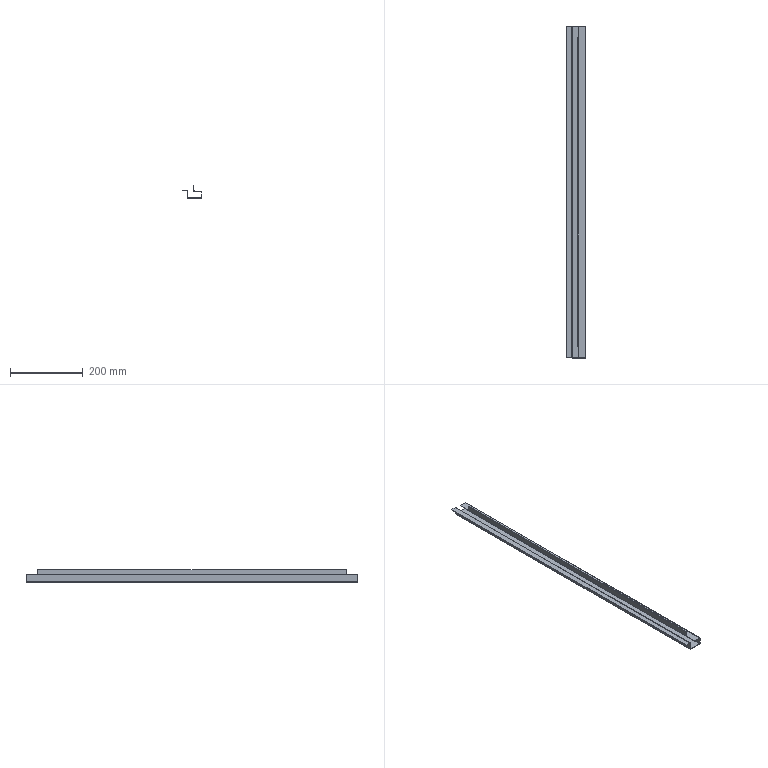Component | SolidWorks | CCQ-1.1-14LowerSidePost1-3 | 1 solid | 46 faces | volume 118197 mm3 | plane 36 | cylinder 10 | commonest cylinder face diameters 3.473 x5 1.473 x5 | material 304